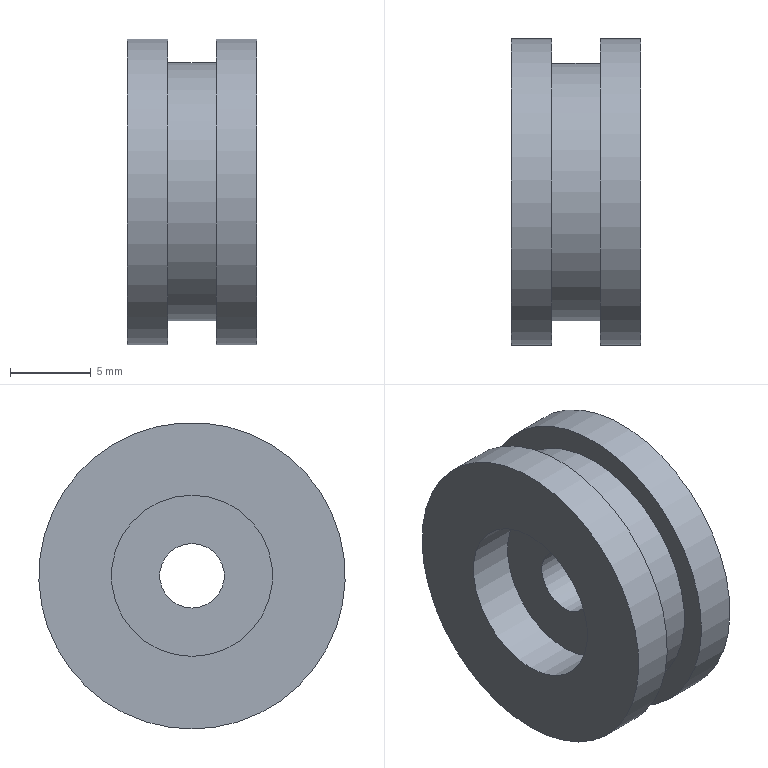Component | NX | PISTON_2 | 1 solid | 10 faces | box 8 x 19 x 19 mm | volume 1722 mm3 | plane 5 | cylinder 5 | commonest cylinder face diameters 19 x2 16 x1 10 x1 4 x1
STEP:
#1=CARTESIAN_POINT('',(0.,0.,0.));
#2=DIRECTION('',(0.,0.,1.));
#3=DIRECTION('',(1.,0.,0.));
#4=AXIS2_PLACEMENT_3D('',#1,#2,#3);
#5=CARTESIAN_POINT('',(-93.299,-36.75,33.));
#6=VERTEX_POINT('',#5);
#7=CARTESIAN_POINT('',(-93.299,-36.75,41.));
#8=DIRECTION('',(1.,0.,0.));
#9=DIRECTION('',(0.,0.,-1.));
#10=AXIS2_PLACEMENT_3D('',#7,#8,#9);
#11=CIRCLE('',#10,8.);
#12=CARTESIAN_POINT('',(-93.299,-36.75,41.));
#13=DIRECTION('',(1.,0.,0.));
#14=DIRECTION('',(0.,0.,-1.));
#15=AXIS2_PLACEMENT_3D('',#12,#13,#14);
#16=PLANE('',#15);
#17=CARTESIAN_POINT('',(0.,0.));
#18=DIRECTION('',(1.,0.));
#19=AXIS2_PLACEMENT_2D('',#17,#18);
#20=CIRCLE('',#19,8.);
#21=(GEOMETRIC_REPRESENTATION_CONTEXT(2)PARAMETRIC_REPRESENTATION_CONTEXT()REPRESENTATION_CONTEXT('',''));
#22=DEFINITIONAL_REPRESENTATION('',(#20),#21);
#23=PCURVE('',#16,#22);
#24=CARTESIAN_POINT('',(-93.299,-36.75,41.));
#25=DIRECTION('',(1.,0.,0.));
#26=DIRECTION('',(0.,0.,-1.));
#27=AXIS2_PLACEMENT_3D('',#24,#25,#26);
#28=CYLINDRICAL_SURFACE('',#27,8.);
#29=CARTESIAN_POINT('',(0.,0.));
#30=DIRECTION('',(1.,0.));
#31=VECTOR('',#30,1.);
#32=LINE('',#29,#31);
#33=(GEOMETRIC_REPRESENTATION_CONTEXT(2)PARAMETRIC_REPRESENTATION_CONTEXT()REPRESENTATION_CONTEXT('',''));
#34=DEFINITIONAL_REPRESENTATION('',(#32),#33);
#35=PCURVE('',#28,#34);
#36=SURFACE_CURVE('',#11,(#23,#35),.PCURVE_S1.);
#37=EDGE_CURVE('',#6,#6,#36,.T.);
#38=ORIENTED_EDGE('',*,*,#37,.F.);
#39=EDGE_LOOP('',(#38));
#40=FACE_BOUND('',#39,.T.);
#41=CARTESIAN_POINT('',(-93.299,-36.75,31.5));
#42=VERTEX_POINT('',#41);
#43=CARTESIAN_POINT('',(-93.299,-36.75,41.));
#44=DIRECTION('',(-1.,0.,0.));
#45=DIRECTION('',(0.,0.,-1.));
#46=AXIS2_PLACEMENT_3D('',#43,#44,#45);
#47=CIRCLE('',#46,9.5);
#48=CARTESIAN_POINT('',(9.5,0.));
#49=CARTESIAN_POINT('',(9.5,-16.454));
#50=CARTESIAN_POINT('',(-4.75,-8.227));
#51=CARTESIAN_POINT('',(-19.,-0.));
#52=CARTESIAN_POINT('',(-4.75,8.227));
#53=CARTESIAN_POINT('',(9.5,16.454));
#54=CARTESIAN_POINT('',(9.5,0.));
#55=(BOUNDED_CURVE()B_SPLINE_CURVE(2,(#48,#49,#50,#51,#52,#53,#54),.UNSPECIFIED.,.T.,.F.)B_SPLINE_CURVE_WITH_KNOTS((1,2,2,2,2,1),(-2.094,0.,2.094,4.189,6.283,8.378),.UNSPECIFIED.)CURVE()GEOMETRIC_REPRESENTATION_ITEM()RATIONAL_B_SPLINE_CURVE((1.,0.5,1.,0.5,1.,0.5,1.))REPRESENTATION_ITEM(''));
#56=(GEOMETRIC_REPRESENTATION_CONTEXT(2)PARAMETRIC_REPRESENTATION_CONTEXT()REPRESENTATION_CONTEXT('',''));
#57=DEFINITIONAL_REPRESENTATION('',(#55),#56);
#58=PCURVE('',#16,#57);
#59=CARTESIAN_POINT('',(-95.799,-36.75,41.));
#60=DIRECTION('',(1.,0.,0.));
#61=DIRECTION('',(0.,0.,-1.));
#62=AXIS2_PLACEMENT_3D('',#59,#60,#61);
#63=CYLINDRICAL_SURFACE('',#62,9.5);
#64=CARTESIAN_POINT('',(6.283,2.5));
#65=DIRECTION('',(-1.,0.));
#66=VECTOR('',#65,1.);
#67=LINE('',#64,#66);
#68=(GEOMETRIC_REPRESENTATION_CONTEXT(2)PARAMETRIC_REPRESENTATION_CONTEXT()REPRESENTATION_CONTEXT('',''));
#69=DEFINITIONAL_REPRESENTATION('',(#67),#68);
#70=PCURVE('',#63,#69);
#71=SURFACE_CURVE('',#47,(#58,#70),.PCURVE_S1.);
#72=EDGE_CURVE('',#42,#42,#71,.T.);
#73=ORIENTED_EDGE('',*,*,#72,.F.);
#74=EDGE_LOOP('',(#73));
#75=FACE_BOUND('',#74,.T.);
#76=ADVANCED_FACE('',(#40,#75),#16,.T.);
#77=CARTESIAN_POINT('',(-95.799,-36.75,36.));
#78=VERTEX_POINT('',#77);
#79=CARTESIAN_POINT('',(-95.799,-36.75,41.));
#80=DIRECTION('',(1.,0.,0.));
#81=DIRECTION('',(0.,0.,-1.));
#82=AXIS2_PLACEMENT_3D('',#79,#80,#81);
#83=CIRCLE('',#82,5.);
#84=CARTESIAN_POINT('',(-95.799,-36.75,41.));
#85=DIRECTION('',(-1.,0.,0.));
#86=DIRECTION('',(0.,0.,1.));
#87=AXIS2_PLACEMENT_3D('',#84,#85,#86);
#88=PLANE('',#87);
#89=CARTESIAN_POINT('',(-5.,0.));
#90=CARTESIAN_POINT('',(-5.,8.66));
#91=CARTESIAN_POINT('',(2.5,4.33));
#92=CARTESIAN_POINT('',(10.,0.));
#93=CARTESIAN_POINT('',(2.5,-4.33));
#94=CARTESIAN_POINT('',(-5.,-8.66));
#95=CARTESIAN_POINT('',(-5.,0.));
#96=(BOUNDED_CURVE()B_SPLINE_CURVE(2,(#89,#90,#91,#92,#93,#94,#95),.UNSPECIFIED.,.T.,.F.)B_SPLINE_CURVE_WITH_KNOTS((1,2,2,2,2,1),(-2.094,0.,2.094,4.189,6.283,8.378),.UNSPECIFIED.)CURVE()GEOMETRIC_REPRESENTATION_ITEM()RATIONAL_B_SPLINE_CURVE((1.,0.5,1.,0.5,1.,0.5,1.))REPRESENTATION_ITEM(''));
#97=(GEOMETRIC_REPRESENTATION_CONTEXT(2)PARAMETRIC_REPRESENTATION_CONTEXT()REPRESENTATION_CONTEXT('',''));
#98=DEFINITIONAL_REPRESENTATION('',(#96),#97);
#99=PCURVE('',#88,#98);
#100=CARTESIAN_POINT('',(-92.799,-36.75,41.));
#101=DIRECTION('',(-1.,0.,0.));
#102=DIRECTION('',(0.,0.,1.));
#103=AXIS2_PLACEMENT_3D('',#100,#101,#102);
#104=CYLINDRICAL_SURFACE('',#103,5.);
#105=CARTESIAN_POINT('',(9.425,3.));
#106=DIRECTION('',(-1.,0.));
#107=VECTOR('',#106,1.);
#108=LINE('',#105,#107);
#109=(GEOMETRIC_REPRESENTATION_CONTEXT(2)PARAMETRIC_REPRESENTATION_CONTEXT()REPRESENTATION_CONTEXT('',''));
#110=DEFINITIONAL_REPRESENTATION('',(#108),#109);
#111=PCURVE('',#104,#110);
#112=SURFACE_CURVE('',#83,(#99,#111),.PCURVE_S1.);
#113=EDGE_CURVE('',#78,#78,#112,.T.);
#114=ORIENTED_EDGE('',*,*,#113,.T.);
#115=EDGE_LOOP('',(#114));
#116=FACE_BOUND('',#115,.T.);
#117=CARTESIAN_POINT('',(-95.799,-36.75,31.5));
#118=VERTEX_POINT('',#117);
#119=CARTESIAN_POINT('',(-95.799,-36.75,41.));
#120=DIRECTION('',(1.,0.,0.));
#121=DIRECTION('',(0.,0.,-1.));
#122=AXIS2_PLACEMENT_3D('',#119,#120,#121);
#123=CIRCLE('',#122,9.5);
#124=CARTESIAN_POINT('',(-9.5,0.));
#125=CARTESIAN_POINT('',(-9.5,16.454));
#126=CARTESIAN_POINT('',(4.75,8.227));
#127=CARTESIAN_POINT('',(19.,0.));
#128=CARTESIAN_POINT('',(4.75,-8.227));
#129=CARTESIAN_POINT('',(-9.5,-16.454));
#130=CARTESIAN_POINT('',(-9.5,0.));
#131=(BOUNDED_CURVE()B_SPLINE_CURVE(2,(#124,#125,#126,#127,#128,#129,#130),.UNSPECIFIED.,.T.,.F.)B_SPLINE_CURVE_WITH_KNOTS((1,2,2,2,2,1),(-2.094,0.,2.094,4.189,6.283,8.378),.UNSPECIFIED.)CURVE()GEOMETRIC_REPRESENTATION_ITEM()RATIONAL_B_SPLINE_CURVE((1.,0.5,1.,0.5,1.,0.5,1.))REPRESENTATION_ITEM(''));
#132=(GEOMETRIC_REPRESENTATION_CONTEXT(2)PARAMETRIC_REPRESENTATION_CONTEXT()REPRESENTATION_CONTEXT('',''));
#133=DEFINITIONAL_REPRESENTATION('',(#131),#132);
#134=PCURVE('',#88,#133);
#135=CARTESIAN_POINT('',(0.,0.));
#136=DIRECTION('',(1.,0.));
#137=VECTOR('',#136,1.);
#138=LINE('',#135,#137);
#139=(GEOMETRIC_REPRESENTATION_CONTEXT(2)PARAMETRIC_REPRESENTATION_CONTEXT()REPRESENTATION_CONTEXT('',''));
#140=DEFINITIONAL_REPRESENTATION('',(#138),#139);
#141=PCURVE('',#63,#140);
#142=SURFACE_CURVE('',#123,(#134,#141),.PCURVE_S1.);
#143=EDGE_CURVE('',#118,#118,#142,.T.);
#144=ORIENTED_EDGE('',*,*,#143,.F.);
#145=EDGE_LOOP('',(#144));
#146=FACE_BOUND('',#145,.T.);
#147=ADVANCED_FACE('',(#116,#146),#88,.T.);
#148=ORIENTED_EDGE('',*,*,#72,.T.);
#149=CARTESIAN_POINT('',(-95.799,-36.75,31.5));
#150=CARTESIAN_POINT('',(-93.299,-36.75,31.5));
#151=B_SPLINE_CURVE_WITH_KNOTS('',1,(#149,#150),.UNSPECIFIED.,.F.,.F.,(2,2),(0.,2.5),.PIECEWISE_BEZIER_KNOTS.);
#152=CARTESIAN_POINT('',(0.,0.));
#153=DIRECTION('',(0.,1.));
#154=VECTOR('',#153,1.);
#155=LINE('',#152,#154);
#156=(GEOMETRIC_REPRESENTATION_CONTEXT(2)PARAMETRIC_REPRESENTATION_CONTEXT()REPRESENTATION_CONTEXT('',''));
#157=DEFINITIONAL_REPRESENTATION('',(#155),#156);
#158=PCURVE('',#63,#157);
#159=CARTESIAN_POINT('',(6.283,0.));
#160=DIRECTION('',(0.,1.));
#161=VECTOR('',#160,1.);
#162=LINE('',#159,#161);
#163=(GEOMETRIC_REPRESENTATION_CONTEXT(2)PARAMETRIC_REPRESENTATION_CONTEXT()REPRESENTATION_CONTEXT('',''));
#164=DEFINITIONAL_REPRESENTATION('',(#162),#163);
#165=PCURVE('',#63,#164);
#166=SEAM_CURVE('',#151,(#158,#165),.PCURVE_S1.);
#167=EDGE_CURVE('',#118,#42,#166,.T.);
#168=ORIENTED_EDGE('',*,*,#167,.F.);
#169=ORIENTED_EDGE('',*,*,#143,.T.);
#170=ORIENTED_EDGE('',*,*,#167,.T.);
#171=EDGE_LOOP('',(#148,#168,#169,#170));
#172=FACE_BOUND('',#171,.T.);
#173=ADVANCED_FACE('',(#172),#63,.T.);
#174=CARTESIAN_POINT('',(-90.299,-36.75,33.));
#175=VERTEX_POINT('',#174);
#176=CARTESIAN_POINT('',(-90.299,-36.75,41.));
#177=DIRECTION('',(1.,0.,0.));
#178=DIRECTION('',(0.,0.,-1.));
#179=AXIS2_PLACEMENT_3D('',#176,#177,#178);
#180=CIRCLE('',#179,8.);
#181=CARTESIAN_POINT('',(0.,3.));
#182=DIRECTION('',(1.,0.));
#183=VECTOR('',#182,1.);
#184=LINE('',#181,#183);
#185=(GEOMETRIC_REPRESENTATION_CONTEXT(2)PARAMETRIC_REPRESENTATION_CONTEXT()REPRESENTATION_CONTEXT('',''));
#186=DEFINITIONAL_REPRESENTATION('',(#184),#185);
#187=PCURVE('',#28,#186);
#188=CARTESIAN_POINT('',(-90.299,-36.75,41.));
#189=DIRECTION('',(-1.,0.,0.));
#190=DIRECTION('',(0.,0.,1.));
#191=AXIS2_PLACEMENT_3D('',#188,#189,#190);
#192=PLANE('',#191);
#193=CARTESIAN_POINT('',(-8.,0.));
#194=CARTESIAN_POINT('',(-8.,13.856));
#195=CARTESIAN_POINT('',(4.,6.928));
#196=CARTESIAN_POINT('',(16.,0.));
#197=CARTESIAN_POINT('',(4.,-6.928));
#198=CARTESIAN_POINT('',(-8.,-13.856));
#199=CARTESIAN_POINT('',(-8.,0.));
#200=(BOUNDED_CURVE()B_SPLINE_CURVE(2,(#193,#194,#195,#196,#197,#198,#199),.UNSPECIFIED.,.T.,.F.)B_SPLINE_CURVE_WITH_KNOTS((1,2,2,2,2,1),(-2.094,0.,2.094,4.189,6.283,8.378),.UNSPECIFIED.)CURVE()GEOMETRIC_REPRESENTATION_ITEM()RATIONAL_B_SPLINE_CURVE((1.,0.5,1.,0.5,1.,0.5,1.))REPRESENTATION_ITEM(''));
#201=(GEOMETRIC_REPRESENTATION_CONTEXT(2)PARAMETRIC_REPRESENTATION_CONTEXT()REPRESENTATION_CONTEXT('',''));
#202=DEFINITIONAL_REPRESENTATION('',(#200),#201);
#203=PCURVE('',#192,#202);
#204=SURFACE_CURVE('',#180,(#187,#203),.PCURVE_S1.);
#205=EDGE_CURVE('',#175,#175,#204,.T.);
#206=ORIENTED_EDGE('',*,*,#205,.F.);
#207=CARTESIAN_POINT('',(-93.299,-36.75,33.));
#208=CARTESIAN_POINT('',(-90.299,-36.75,33.));
#209=B_SPLINE_CURVE_WITH_KNOTS('',1,(#207,#208),.UNSPECIFIED.,.F.,.F.,(2,2),(0.,3.),.PIECEWISE_BEZIER_KNOTS.);
#210=CARTESIAN_POINT('',(0.,0.));
#211=DIRECTION('',(0.,1.));
#212=VECTOR('',#211,1.);
#213=LINE('',#210,#212);
#214=(GEOMETRIC_REPRESENTATION_CONTEXT(2)PARAMETRIC_REPRESENTATION_CONTEXT()REPRESENTATION_CONTEXT('',''));
#215=DEFINITIONAL_REPRESENTATION('',(#213),#214);
#216=PCURVE('',#28,#215);
#217=CARTESIAN_POINT('',(6.283,0.));
#218=DIRECTION('',(0.,1.));
#219=VECTOR('',#218,1.);
#220=LINE('',#217,#219);
#221=(GEOMETRIC_REPRESENTATION_CONTEXT(2)PARAMETRIC_REPRESENTATION_CONTEXT()REPRESENTATION_CONTEXT('',''));
#222=DEFINITIONAL_REPRESENTATION('',(#220),#221);
#223=PCURVE('',#28,#222);
#224=SEAM_CURVE('',#209,(#216,#223),.PCURVE_S1.);
#225=EDGE_CURVE('',#6,#175,#224,.T.);
#226=ORIENTED_EDGE('',*,*,#225,.F.);
#227=ORIENTED_EDGE('',*,*,#37,.T.);
#228=ORIENTED_EDGE('',*,*,#225,.T.);
#229=EDGE_LOOP('',(#206,#226,#227,#228));
#230=FACE_BOUND('',#229,.T.);
#231=ADVANCED_FACE('',(#230),#28,.T.);
#232=CARTESIAN_POINT('',(-87.799,-36.75,39.));
#233=VERTEX_POINT('',#232);
#234=CARTESIAN_POINT('',(-87.799,-36.75,41.));
#235=DIRECTION('',(1.,0.,0.));
#236=DIRECTION('',(0.,0.,-1.));
#237=AXIS2_PLACEMENT_3D('',#234,#235,#236);
#238=CIRCLE('',#237,2.);
#239=CARTESIAN_POINT('',(-87.799,-36.75,41.));
#240=DIRECTION('',(1.,0.,0.));
#241=DIRECTION('',(0.,0.,-1.));
#242=AXIS2_PLACEMENT_3D('',#239,#240,#241);
#243=PLANE('',#242);
#244=CARTESIAN_POINT('',(0.,0.));
#245=DIRECTION('',(1.,0.));
#246=AXIS2_PLACEMENT_2D('',#244,#245);
#247=CIRCLE('',#246,2.);
#248=(GEOMETRIC_REPRESENTATION_CONTEXT(2)PARAMETRIC_REPRESENTATION_CONTEXT()REPRESENTATION_CONTEXT('',''));
#249=DEFINITIONAL_REPRESENTATION('',(#247),#248);
#250=PCURVE('',#243,#249);
#251=CARTESIAN_POINT('',(-92.799,-36.75,41.));
#252=DIRECTION('',(1.,0.,0.));
#253=DIRECTION('',(0.,0.,-1.));
#254=AXIS2_PLACEMENT_3D('',#251,#252,#253);
#255=CYLINDRICAL_SURFACE('',#254,2.);
#256=CARTESIAN_POINT('',(0.,5.));
#257=DIRECTION('',(1.,0.));
#258=VECTOR('',#257,1.);
#259=LINE('',#256,#258);
#260=(GEOMETRIC_REPRESENTATION_CONTEXT(2)PARAMETRIC_REPRESENTATION_CONTEXT()REPRESENTATION_CONTEXT('',''));
#261=DEFINITIONAL_REPRESENTATION('',(#259),#260);
#262=PCURVE('',#255,#261);
#263=SURFACE_CURVE('',#238,(#250,#262),.PCURVE_S1.);
#264=EDGE_CURVE('',#233,#233,#263,.T.);
#265=ORIENTED_EDGE('',*,*,#264,.F.);
#266=EDGE_LOOP('',(#265));
#267=FACE_BOUND('',#266,.T.);
#268=CARTESIAN_POINT('',(-87.799,-36.75,31.5));
#269=VERTEX_POINT('',#268);
#270=CARTESIAN_POINT('',(-87.799,-36.75,41.));
#271=DIRECTION('',(1.,0.,0.));
#272=DIRECTION('',(0.,0.,-1.));
#273=AXIS2_PLACEMENT_3D('',#270,#271,#272);
#274=CIRCLE('',#273,9.5);
#275=CARTESIAN_POINT('',(0.,0.));
#276=DIRECTION('',(1.,0.));
#277=AXIS2_PLACEMENT_2D('',#275,#276);
#278=CIRCLE('',#277,9.5);
#279=(GEOMETRIC_REPRESENTATION_CONTEXT(2)PARAMETRIC_REPRESENTATION_CONTEXT()REPRESENTATION_CONTEXT('',''));
#280=DEFINITIONAL_REPRESENTATION('',(#278),#279);
#281=PCURVE('',#243,#280);
#282=CARTESIAN_POINT('',(-90.299,-36.75,41.));
#283=DIRECTION('',(1.,0.,0.));
#284=DIRECTION('',(0.,0.,-1.));
#285=AXIS2_PLACEMENT_3D('',#282,#283,#284);
#286=CYLINDRICAL_SURFACE('',#285,9.5);
#287=CARTESIAN_POINT('',(0.,2.5));
#288=DIRECTION('',(1.,0.));
#289=VECTOR('',#288,1.);
#290=LINE('',#287,#289);
#291=(GEOMETRIC_REPRESENTATION_CONTEXT(2)PARAMETRIC_REPRESENTATION_CONTEXT()REPRESENTATION_CONTEXT('',''));
#292=DEFINITIONAL_REPRESENTATION('',(#290),#291);
#293=PCURVE('',#286,#292);
#294=SURFACE_CURVE('',#274,(#281,#293),.PCURVE_S1.);
#295=EDGE_CURVE('',#269,#269,#294,.T.);
#296=ORIENTED_EDGE('',*,*,#295,.T.);
#297=EDGE_LOOP('',(#296));
#298=FACE_BOUND('',#297,.T.);
#299=ADVANCED_FACE('',(#267,#298),#243,.T.);
#300=ORIENTED_EDGE('',*,*,#205,.T.);
#301=EDGE_LOOP('',(#300));
#302=FACE_BOUND('',#301,.T.);
#303=CARTESIAN_POINT('',(-90.299,-36.75,31.5));
#304=VERTEX_POINT('',#303);
#305=CARTESIAN_POINT('',(-90.299,-36.75,41.));
#306=DIRECTION('',(1.,0.,0.));
#307=DIRECTION('',(0.,0.,-1.));
#308=AXIS2_PLACEMENT_3D('',#305,#306,#307);
#309=CIRCLE('',#308,9.5);
#310=CARTESIAN_POINT('',(-9.5,0.));
#311=CARTESIAN_POINT('',(-9.5,16.454));
#312=CARTESIAN_POINT('',(4.75,8.227));
#313=CARTESIAN_POINT('',(19.,0.));
#314=CARTESIAN_POINT('',(4.75,-8.227));
#315=CARTESIAN_POINT('',(-9.5,-16.454));
#316=CARTESIAN_POINT('',(-9.5,0.));
#317=(BOUNDED_CURVE()B_SPLINE_CURVE(2,(#310,#311,#312,#313,#314,#315,#316),.UNSPECIFIED.,.T.,.F.)B_SPLINE_CURVE_WITH_KNOTS((1,2,2,2,2,1),(-2.094,0.,2.094,4.189,6.283,8.378),.UNSPECIFIED.)CURVE()GEOMETRIC_REPRESENTATION_ITEM()RATIONAL_B_SPLINE_CURVE((1.,0.5,1.,0.5,1.,0.5,1.))REPRESENTATION_ITEM(''));
#318=(GEOMETRIC_REPRESENTATION_CONTEXT(2)PARAMETRIC_REPRESENTATION_CONTEXT()REPRESENTATION_CONTEXT('',''));
#319=DEFINITIONAL_REPRESENTATION('',(#317),#318);
#320=PCURVE('',#192,#319);
#321=CARTESIAN_POINT('',(0.,0.));
#322=DIRECTION('',(1.,0.));
#323=VECTOR('',#322,1.);
#324=LINE('',#321,#323);
#325=(GEOMETRIC_REPRESENTATION_CONTEXT(2)PARAMETRIC_REPRESENTATION_CONTEXT()REPRESENTATION_CONTEXT('',''));
#326=DEFINITIONAL_REPRESENTATION('',(#324),#325);
#327=PCURVE('',#286,#326);
#328=SURFACE_CURVE('',#309,(#320,#327),.PCURVE_S1.);
#329=EDGE_CURVE('',#304,#304,#328,.T.);
#330=ORIENTED_EDGE('',*,*,#329,.F.);
#331=EDGE_LOOP('',(#330));
#332=FACE_BOUND('',#331,.T.);
#333=ADVANCED_FACE('',(#302,#332),#192,.T.);
#334=ORIENTED_EDGE('',*,*,#295,.F.);
#335=CARTESIAN_POINT('',(-90.299,-36.75,31.5));
#336=CARTESIAN_POINT('',(-87.799,-36.75,31.5));
#337=B_SPLINE_CURVE_WITH_KNOTS('',1,(#335,#336),.UNSPECIFIED.,.F.,.F.,(2,2),(0.,2.5),.PIECEWISE_BEZIER_KNOTS.);
#338=CARTESIAN_POINT('',(0.,0.));
#339=DIRECTION('',(0.,1.));
#340=VECTOR('',#339,1.);
#341=LINE('',#338,#340);
#342=(GEOMETRIC_REPRESENTATION_CONTEXT(2)PARAMETRIC_REPRESENTATION_CONTEXT()REPRESENTATION_CONTEXT('',''));
#343=DEFINITIONAL_REPRESENTATION('',(#341),#342);
#344=PCURVE('',#286,#343);
#345=CARTESIAN_POINT('',(6.283,0.));
#346=DIRECTION('',(0.,1.));
#347=VECTOR('',#346,1.);
#348=LINE('',#345,#347);
#349=(GEOMETRIC_REPRESENTATION_CONTEXT(2)PARAMETRIC_REPRESENTATION_CONTEXT()REPRESENTATION_CONTEXT('',''));
#350=DEFINITIONAL_REPRESENTATION('',(#348),#349);
#351=PCURVE('',#286,#350);
#352=SEAM_CURVE('',#337,(#344,#351),.PCURVE_S1.);
#353=EDGE_CURVE('',#304,#269,#352,.T.);
#354=ORIENTED_EDGE('',*,*,#353,.F.);
#355=ORIENTED_EDGE('',*,*,#329,.T.);
#356=ORIENTED_EDGE('',*,*,#353,.T.);
#357=EDGE_LOOP('',(#334,#354,#355,#356));
#358=FACE_BOUND('',#357,.T.);
#359=ADVANCED_FACE('',(#358),#286,.T.);
#360=CARTESIAN_POINT('',(-92.799,-36.75,36.));
#361=VERTEX_POINT('',#360);
#362=CARTESIAN_POINT('',(-92.799,-36.75,41.));
#363=DIRECTION('',(-1.,0.,0.));
#364=DIRECTION('',(0.,0.,-1.));
#365=AXIS2_PLACEMENT_3D('',#362,#363,#364);
#366=CIRCLE('',#365,5.);
#367=CARTESIAN_POINT('',(3.142,0.));
#368=DIRECTION('',(1.,0.));
#369=VECTOR('',#368,1.);
#370=LINE('',#367,#369);
#371=(GEOMETRIC_REPRESENTATION_CONTEXT(2)PARAMETRIC_REPRESENTATION_CONTEXT()REPRESENTATION_CONTEXT('',''));
#372=DEFINITIONAL_REPRESENTATION('',(#370),#371);
#373=PCURVE('',#104,#372);
#374=CARTESIAN_POINT('',(-92.799,-36.75,41.));
#375=DIRECTION('',(1.,0.,0.));
#376=DIRECTION('',(0.,0.,-1.));
#377=AXIS2_PLACEMENT_3D('',#374,#375,#376);
#378=PLANE('',#377);
#379=CARTESIAN_POINT('',(5.,0.));
#380=CARTESIAN_POINT('',(5.,-8.66));
#381=CARTESIAN_POINT('',(-2.5,-4.33));
#382=CARTESIAN_POINT('',(-10.,-0.));
#383=CARTESIAN_POINT('',(-2.5,4.33));
#384=CARTESIAN_POINT('',(5.,8.66));
#385=CARTESIAN_POINT('',(5.,0.));
#386=(BOUNDED_CURVE()B_SPLINE_CURVE(2,(#379,#380,#381,#382,#383,#384,#385),.UNSPECIFIED.,.T.,.F.)B_SPLINE_CURVE_WITH_KNOTS((1,2,2,2,2,1),(-2.094,0.,2.094,4.189,6.283,8.378),.UNSPECIFIED.)CURVE()GEOMETRIC_REPRESENTATION_ITEM()RATIONAL_B_SPLINE_CURVE((1.,0.5,1.,0.5,1.,0.5,1.))REPRESENTATION_ITEM(''));
#387=(GEOMETRIC_REPRESENTATION_CONTEXT(2)PARAMETRIC_REPRESENTATION_CONTEXT()REPRESENTATION_CONTEXT('',''));
#388=DEFINITIONAL_REPRESENTATION('',(#386),#387);
#389=PCURVE('',#378,#388);
#390=SURFACE_CURVE('',#366,(#373,#389),.PCURVE_S1.);
#391=EDGE_CURVE('',#361,#361,#390,.T.);
#392=ORIENTED_EDGE('',*,*,#391,.T.);
#393=CARTESIAN_POINT('',(-92.799,-36.75,36.));
#394=CARTESIAN_POINT('',(-95.799,-36.75,36.));
#395=B_SPLINE_CURVE_WITH_KNOTS('',1,(#393,#394),.UNSPECIFIED.,.F.,.F.,(2,2),(0.,3.),.PIECEWISE_BEZIER_KNOTS.);
#396=CARTESIAN_POINT('',(9.425,0.));
#397=DIRECTION('',(0.,1.));
#398=VECTOR('',#397,1.);
#399=LINE('',#396,#398);
#400=(GEOMETRIC_REPRESENTATION_CONTEXT(2)PARAMETRIC_REPRESENTATION_CONTEXT()REPRESENTATION_CONTEXT('',''));
#401=DEFINITIONAL_REPRESENTATION('',(#399),#400);
#402=PCURVE('',#104,#401);
#403=CARTESIAN_POINT('',(3.142,0.));
#404=DIRECTION('',(0.,1.));
#405=VECTOR('',#404,1.);
#406=LINE('',#403,#405);
#407=(GEOMETRIC_REPRESENTATION_CONTEXT(2)PARAMETRIC_REPRESENTATION_CONTEXT()REPRESENTATION_CONTEXT('',''));
#408=DEFINITIONAL_REPRESENTATION('',(#406),#407);
#409=PCURVE('',#104,#408);
#410=SEAM_CURVE('',#395,(#402,#409),.PCURVE_S1.);
#411=EDGE_CURVE('',#361,#78,#410,.T.);
#412=ORIENTED_EDGE('',*,*,#411,.T.);
#413=ORIENTED_EDGE('',*,*,#113,.T.);
#414=ORIENTED_EDGE('',*,*,#411,.F.);
#415=EDGE_LOOP('',(#392,#412,#413,#414));
#416=FACE_BOUND('',#415,.F.);
#417=ADVANCED_FACE('',(#416),#104,.F.);
#418=CARTESIAN_POINT('',(-92.799,-36.75,39.));
#419=VERTEX_POINT('',#418);
#420=CARTESIAN_POINT('',(-92.799,-36.75,41.));
#421=DIRECTION('',(1.,0.,0.));
#422=DIRECTION('',(0.,0.,-1.));
#423=AXIS2_PLACEMENT_3D('',#420,#421,#422);
#424=CIRCLE('',#423,2.);
#425=CARTESIAN_POINT('',(0.,0.));
#426=DIRECTION('',(1.,0.));
#427=AXIS2_PLACEMENT_2D('',#425,#426);
#428=CIRCLE('',#427,2.);
#429=(GEOMETRIC_REPRESENTATION_CONTEXT(2)PARAMETRIC_REPRESENTATION_CONTEXT()REPRESENTATION_CONTEXT('',''));
#430=DEFINITIONAL_REPRESENTATION('',(#428),#429);
#431=PCURVE('',#378,#430);
#432=CARTESIAN_POINT('',(0.,0.));
#433=DIRECTION('',(1.,0.));
#434=VECTOR('',#433,1.);
#435=LINE('',#432,#434);
#436=(GEOMETRIC_REPRESENTATION_CONTEXT(2)PARAMETRIC_REPRESENTATION_CONTEXT()REPRESENTATION_CONTEXT('',''));
#437=DEFINITIONAL_REPRESENTATION('',(#435),#436);
#438=PCURVE('',#255,#437);
#439=SURFACE_CURVE('',#424,(#431,#438),.PCURVE_S1.);
#440=EDGE_CURVE('',#419,#419,#439,.T.);
#441=ORIENTED_EDGE('',*,*,#440,.T.);
#442=EDGE_LOOP('',(#441));
#443=FACE_BOUND('',#442,.T.);
#444=ORIENTED_EDGE('',*,*,#391,.T.);
#445=EDGE_LOOP('',(#444));
#446=FACE_BOUND('',#445,.T.);
#447=ADVANCED_FACE('',(#443,#446),#378,.F.);
#448=ORIENTED_EDGE('',*,*,#264,.F.);
#449=CARTESIAN_POINT('',(-92.799,-36.75,39.));
#450=CARTESIAN_POINT('',(-87.799,-36.75,39.));
#451=B_SPLINE_CURVE_WITH_KNOTS('',1,(#449,#450),.UNSPECIFIED.,.F.,.F.,(2,2),(0.,5.),.PIECEWISE_BEZIER_KNOTS.);
#452=CARTESIAN_POINT('',(0.,0.));
#453=DIRECTION('',(0.,1.));
#454=VECTOR('',#453,1.);
#455=LINE('',#452,#454);
#456=(GEOMETRIC_REPRESENTATION_CONTEXT(2)PARAMETRIC_REPRESENTATION_CONTEXT()REPRESENTATION_CONTEXT('',''));
#457=DEFINITIONAL_REPRESENTATION('',(#455),#456);
#458=PCURVE('',#255,#457);
#459=CARTESIAN_POINT('',(6.283,0.));
#460=DIRECTION('',(0.,1.));
#461=VECTOR('',#460,1.);
#462=LINE('',#459,#461);
#463=(GEOMETRIC_REPRESENTATION_CONTEXT(2)PARAMETRIC_REPRESENTATION_CONTEXT()REPRESENTATION_CONTEXT('',''));
#464=DEFINITIONAL_REPRESENTATION('',(#462),#463);
#465=PCURVE('',#255,#464);
#466=SEAM_CURVE('',#451,(#458,#465),.PCURVE_S1.);
#467=EDGE_CURVE('',#419,#233,#466,.T.);
#468=ORIENTED_EDGE('',*,*,#467,.F.);
#469=ORIENTED_EDGE('',*,*,#440,.T.);
#470=ORIENTED_EDGE('',*,*,#467,.T.);
#471=EDGE_LOOP('',(#448,#468,#469,#470));
#472=FACE_BOUND('',#471,.F.);
#473=ADVANCED_FACE('',(#472),#255,.F.);
#474=CLOSED_SHELL('',(#76,#147,#173,#231,#299,#333,#359,#417,#447,#473));
#475=MANIFOLD_SOLID_BREP('',#474);
#476=(LENGTH_UNIT()NAMED_UNIT(*)SI_UNIT(.MILLI.,.METRE.));
#477=UNCERTAINTY_MEASURE_WITH_UNIT(LENGTH_MEASURE(0.00001),#476,'','');
#478=(NAMED_UNIT(*)PLANE_ANGLE_UNIT()SI_UNIT($,.RADIAN.));
#479=(NAMED_UNIT(*)SI_UNIT($,.STERADIAN.)SOLID_ANGLE_UNIT());
#480=(GEOMETRIC_REPRESENTATION_CONTEXT(3)GLOBAL_UNCERTAINTY_ASSIGNED_CONTEXT((#477))GLOBAL_UNIT_ASSIGNED_CONTEXT((#476,#478,#479))REPRESENTATION_CONTEXT('',''));
#481=ADVANCED_BREP_SHAPE_REPRESENTATION('',(#4,#475),#480);